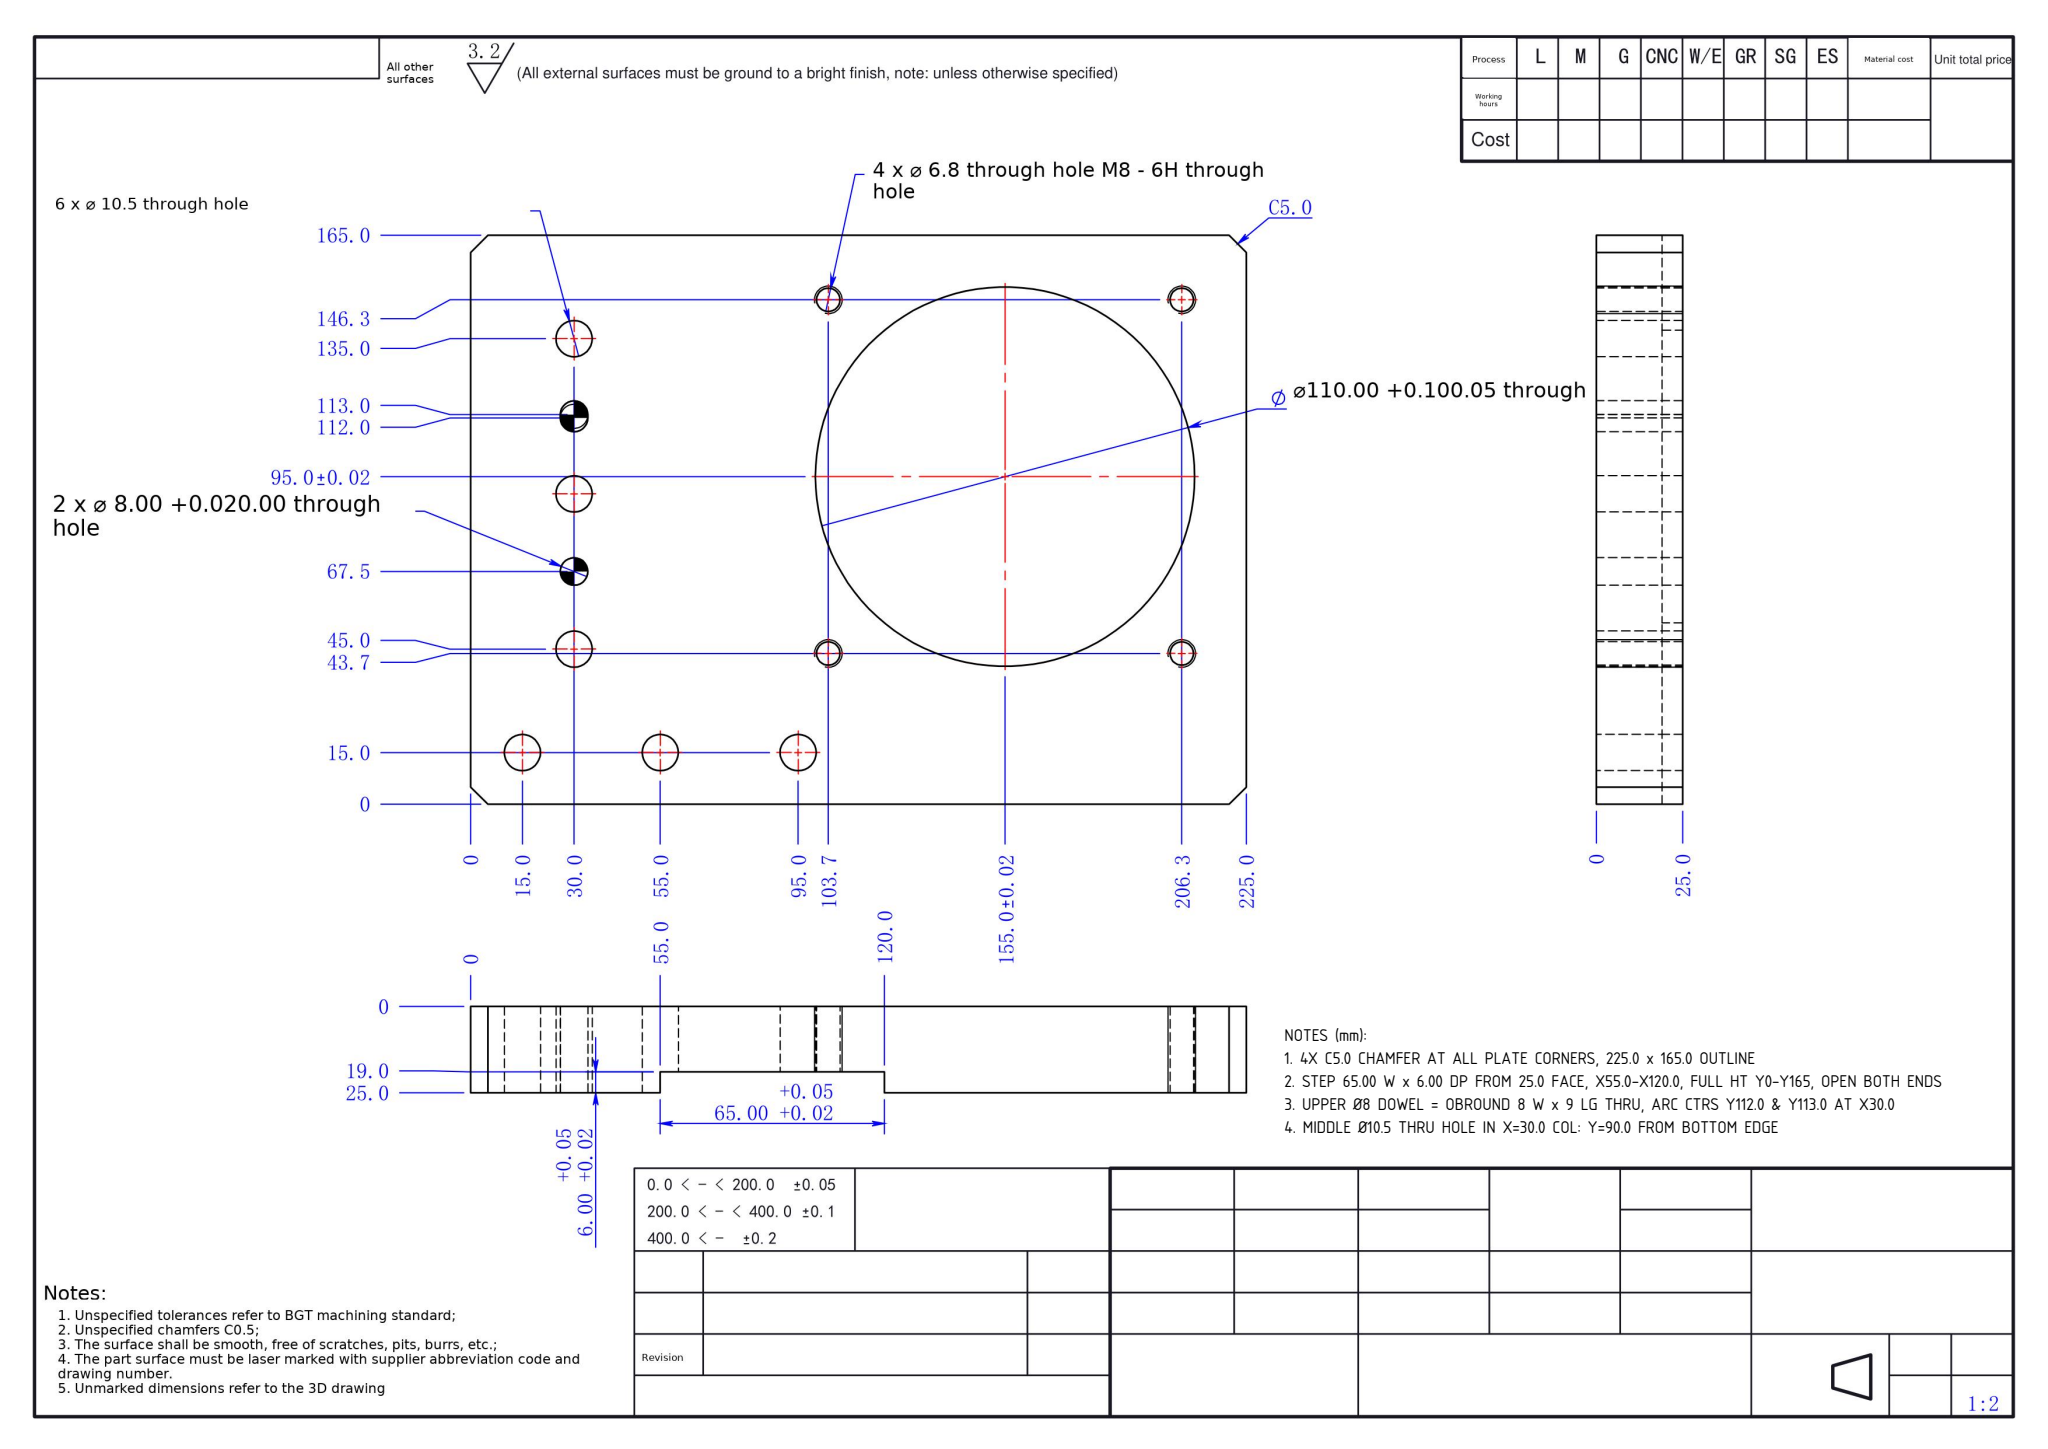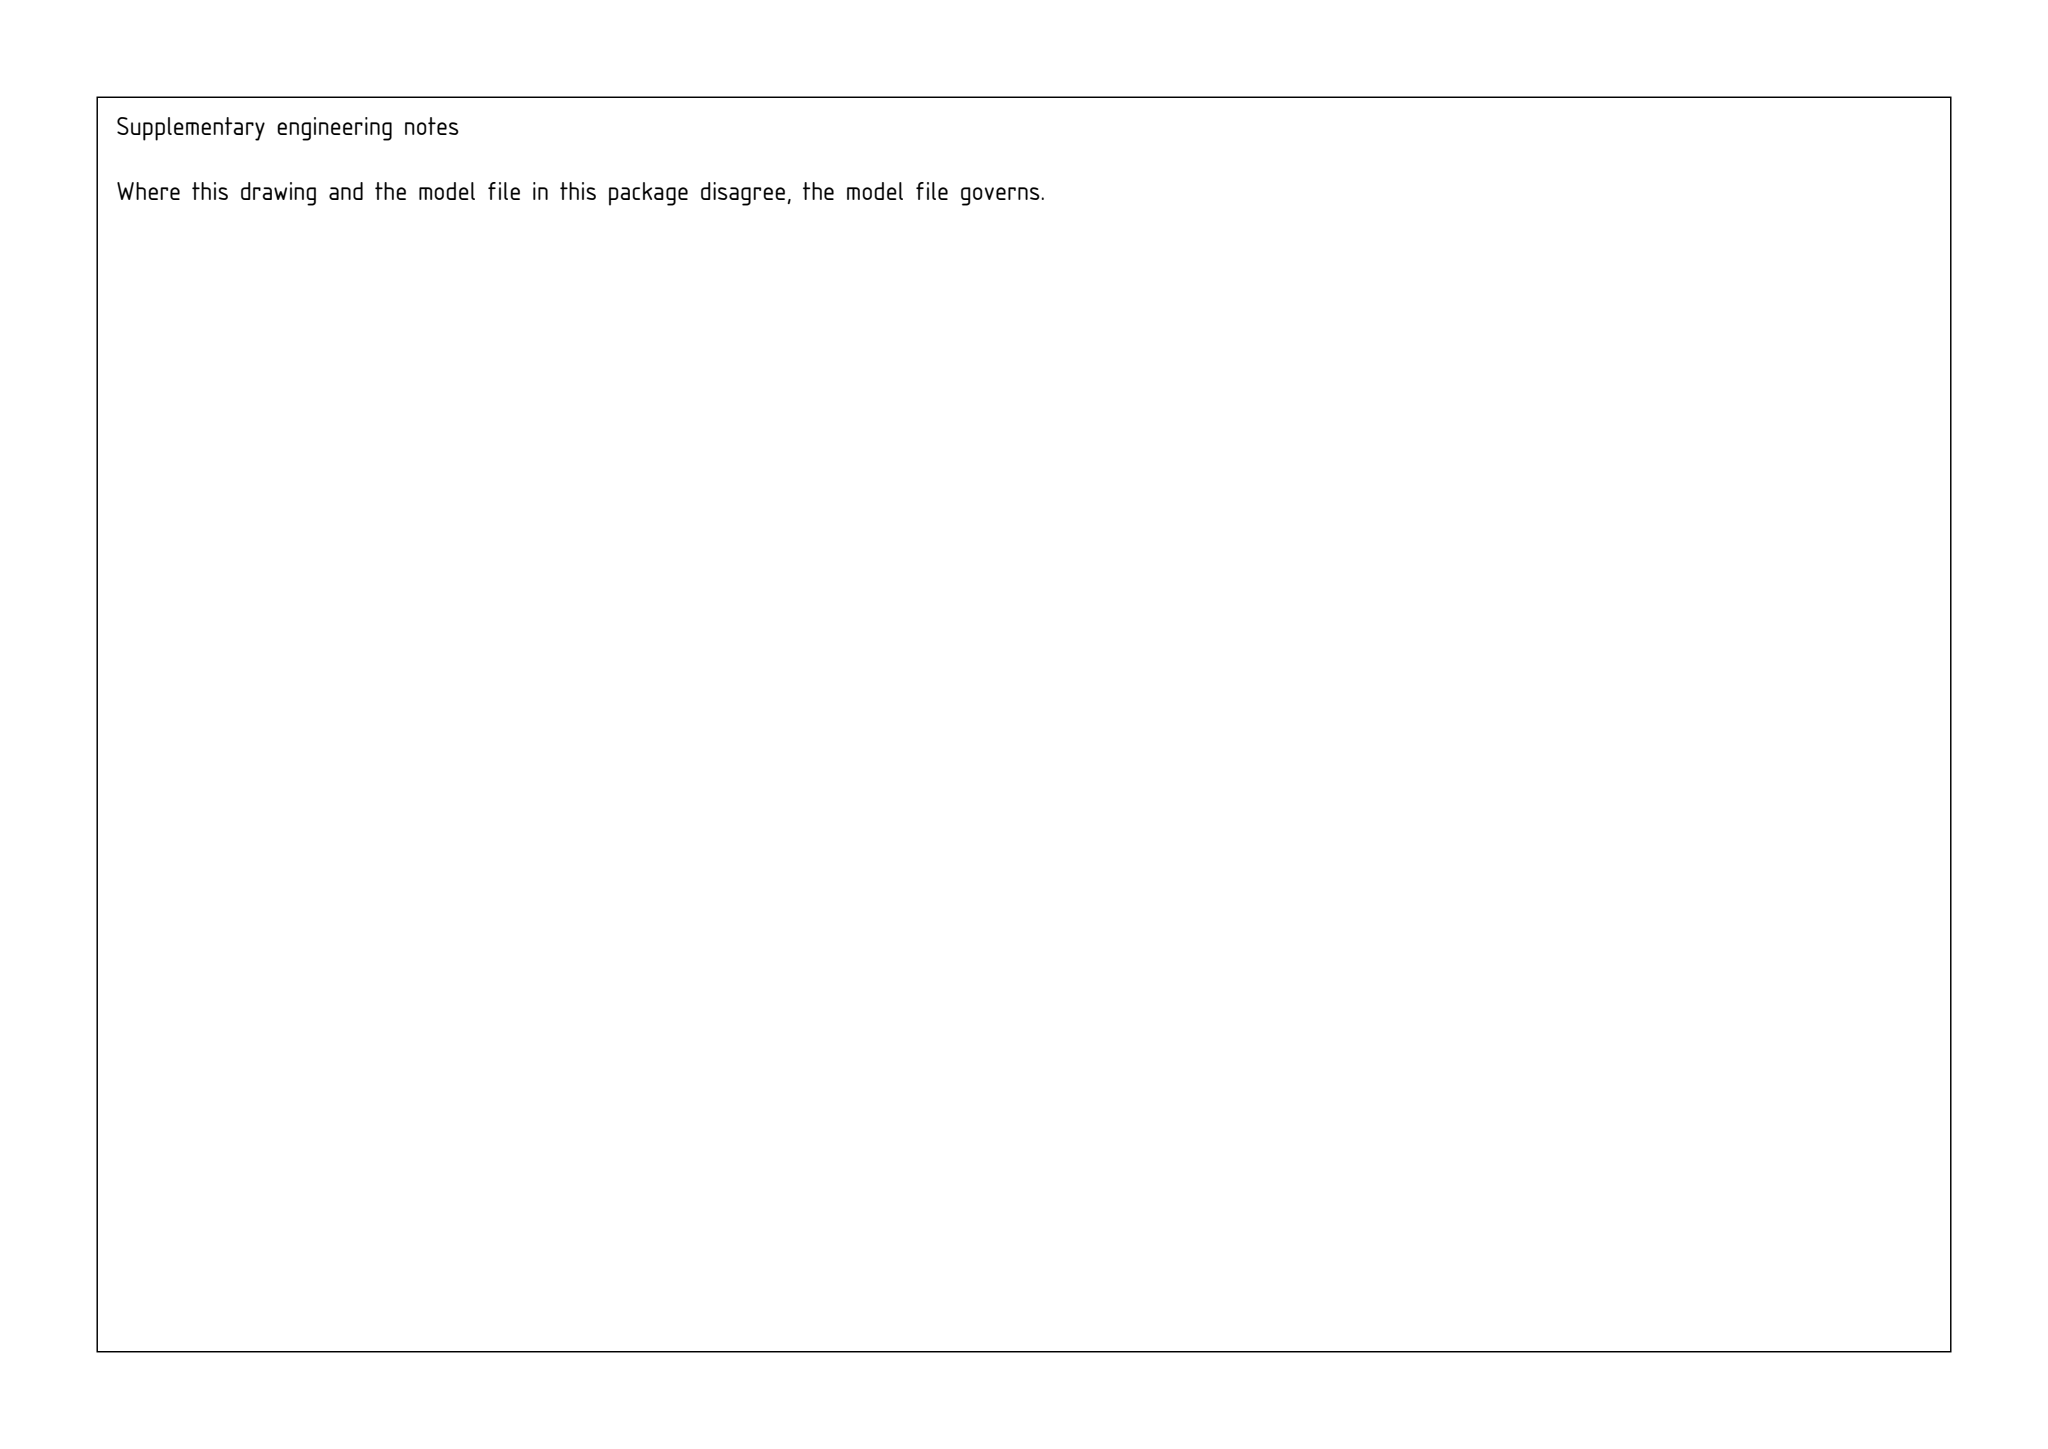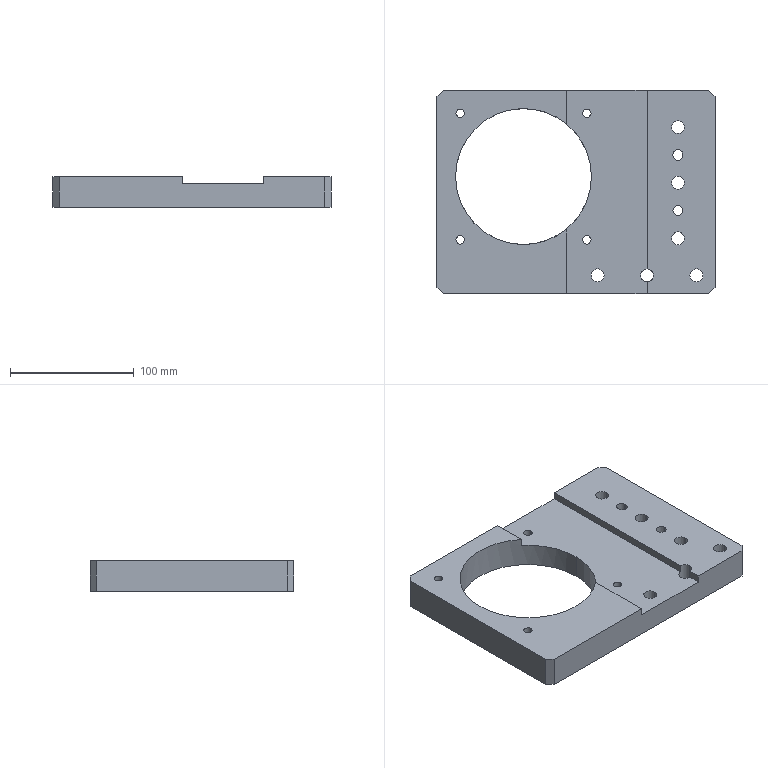Part | SolidWorks | mm | 1 solid | 44 faces | box 225 x 165 x 25 mm | volume 613905 mm3 | cylinder 26 | plane 18 | commonest cylinder face diameters 10.5 x12 6.8 x8 8 x4 110 x2
Drawing notes:
4X C5.0 CHAMFER AT ALL PLATE CORNERS, 225.0 x 165.0 OUTLINE | from the solid: Plate bbox 225.0 x 165.0 x 25.0, no fillet radii; all four top-view corners broken equally, one C5.0 callout
STEP 65.00 W x 6.00 DP FROM 25.0 FACE, X55.0-X120.0, FULL HT Y0-Y165, OPEN BOTH ENDS | from the solid: z planes 0/19.0/25.0 (25-19=6); x planes 105.0 & 170.0 = drawing 55.0 & 120.0; only y planes 0.0 and 165.0, no y walls bound the step
UPPER Ø8 DOWEL = OBROUND 8 W x 9 LG THRU, ARC CTRS Y112.0 & Y113.0 AT X30.0 | from the solid: Ø8 half-cyl faces at x=195 with y=112.0 and y=113.0, length 25 thru; drawing X = 225 - 195 = 30.0
MIDDLE Ø10.5 THRU HOLE IN X=30.0 COL: Y=90.0 FROM BOTTOM EDGE | from the solid: cylinder dia 10.5, axis z, pos [195.0, 90.0], length 25.0; bbox Y=165.0, X=225.0 (drawing X=225-195=30.0)
build123d program:
from build123d import *

# Parameters (mm, degrees)
SKETCH1_W                    = 225
SKETCH1_H                    = 135
BOSS_EXTRUDE1_DEPTH          = 25
SKETCH7_W                    = 120
SKETCH7_H                    = 25
BOSS_EXTRUDE2_DEPTH          = 30
SKETCH8_W                    = 105
SKETCH8_H                    = 25
BOSS_EXTRUDE3_DEPTH          = 30
CHAMFER2_SIZE                = 5
SKETCH2_R                    = 55
CUT_EXTRUDE1_DEPTH           = 151.955
M8_TAPPED_HOLE1_D            = 6.8
F_10_5_10_5_DIAMETER_HOLE1_D = 10.5
SKETCH10_W                   = 65
SKETCH10_H                   = 6
CUT_EXTRUDE2_DEPTH           = 202.262
SIZE_MM_DOWEL_PIN_HOLE1_D    = 8
CUT_EXTRUDE3_DEPTH           = 151.955


with BuildPart() as part:
    # Sketch1 → Boss-Extrude1 (new body)
    with BuildSketch(Plane.XY):
        Rectangle(SKETCH1_W, SKETCH1_H)
    extrude(amount=BOSS_EXTRUDE1_DEPTH)

    # Sketch7 → Boss-Extrude2 (add)
    with BuildSketch(Plane.XZ.offset(67.5)):
        with Locations((52.5, 12.5)):
            Rectangle(SKETCH7_W, SKETCH7_H)
    extrude(amount=BOSS_EXTRUDE2_DEPTH)

    # Sketch8 → Boss-Extrude3 (add)
    with BuildSketch(Plane.XZ.offset(67.5)):
        with Locations((-60, 12.5)):
            Rectangle(SKETCH8_W, SKETCH8_H)
    extrude(amount=BOSS_EXTRUDE3_DEPTH)

    # Chamfer2
    chamfer2_edges = [part.edges().sort_by_distance(p)[0] for p in [
        (112.5, -97.5, 12.5),
        (-112.5, -97.5, 12.5),
        (-112.5, 67.5, 12.5),
        (112.5, 67.5, 12.5),
    ]]
    chamfer(chamfer2_edges, length=CHAMFER2_SIZE)

    # Sketch2 → Cut-Extrude1 (cut, through all)
    with BuildSketch(Plane(origin=(0, 0, 0), x_dir=(-1, 0, 0), z_dir=(0, 0, -1))):
        with Locations((42.5, -2.5)):
            Circle(SKETCH2_R)
    extrude(amount=-CUT_EXTRUDE1_DEPTH, mode=Mode.SUBTRACT)

    # M8 Tapped Hole1 (through all)
    with Locations(Plane(origin=(0, 0, 0), x_dir=(-1, 0, 0), z_dir=(0, 0, -1))):
        with Locations((-8.765, 48.765), (93.765, 48.765), (-8.765, -53.765), (93.765, -53.765)):
            Hole(M8_TAPPED_HOLE1_D / 2)

    # 10.5 _10.5_ Diameter Hole1 (through all)
    with Locations(Plane.XY.offset(25)):
        with Locations((82.5, 37.5), (82.5, -7.5), (82.5, -52.5), (97.5, -82.5), (57.5, -82.5), (17.5, -82.5)):
            Hole(F_10_5_10_5_DIAMETER_HOLE1_D / 2)

    # Sketch10 → Cut-Extrude2 (cut, through all)
    with BuildSketch(Plane(origin=(0, 67.5, 0), x_dir=(1, 0, 0), z_dir=(0, 1, 0))):
        with Locations((25, -22)):
            Rectangle(SKETCH10_W, SKETCH10_H)
    extrude(amount=-CUT_EXTRUDE2_DEPTH, mode=Mode.SUBTRACT)

    # Size mm Dowel Pin Hole1 (through all)
    with Locations(Plane(origin=(0, 0, 0), x_dir=(-1, 0, 0), z_dir=(0, 0, -1))):
        with Locations((-82.5, -30), (-82.5, 15)):
            Hole(SIZE_MM_DOWEL_PIN_HOLE1_D / 2)

    # Sketch14 → Cut-Extrude3 (cut, through all)
    with BuildSketch(Plane(origin=(0, 0, 0), x_dir=(-1, 0, 0), z_dir=(0, 0, -1))):
        with BuildLine():
            Line((-86.5, 14.5), (-86.5, 15.5))
            ThreePointArc((-86.5, 15.5), (-82.5, 19.5), (-78.5, 15.5))
            Line((-78.5, 15.5), (-78.5, 14.5))
            ThreePointArc((-78.5, 14.5), (-82.5, 10.5), (-86.5, 14.5))
        make_face()
    extrude(amount=-CUT_EXTRUDE3_DEPTH, mode=Mode.SUBTRACT)


solid = part.part